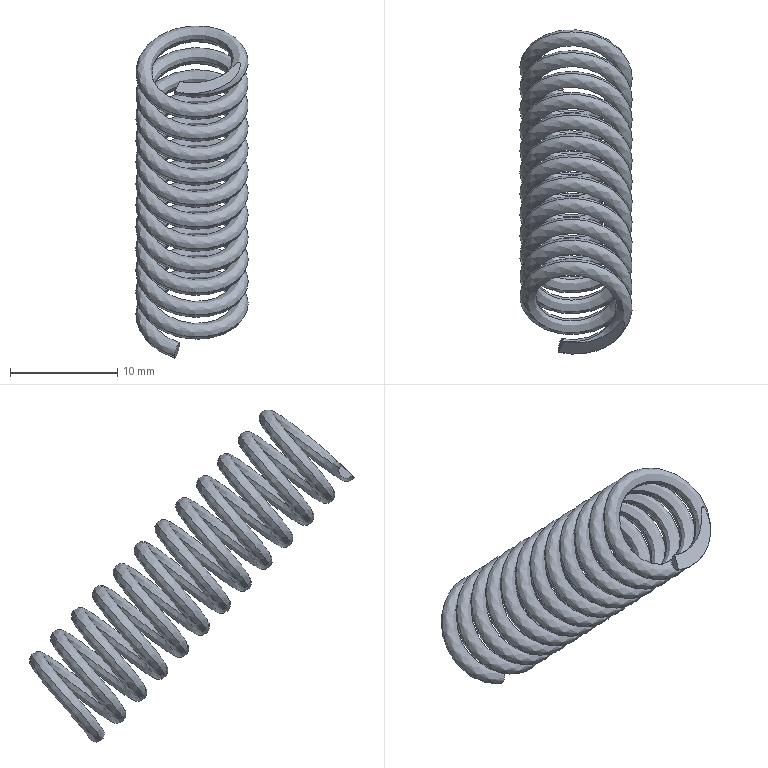Component | SolidWorks | SeedingAssemblyA-1_DuckbillSpring-10 | 1 solid | 5 faces | volume 599 mm3 | plane 3 | spline 2